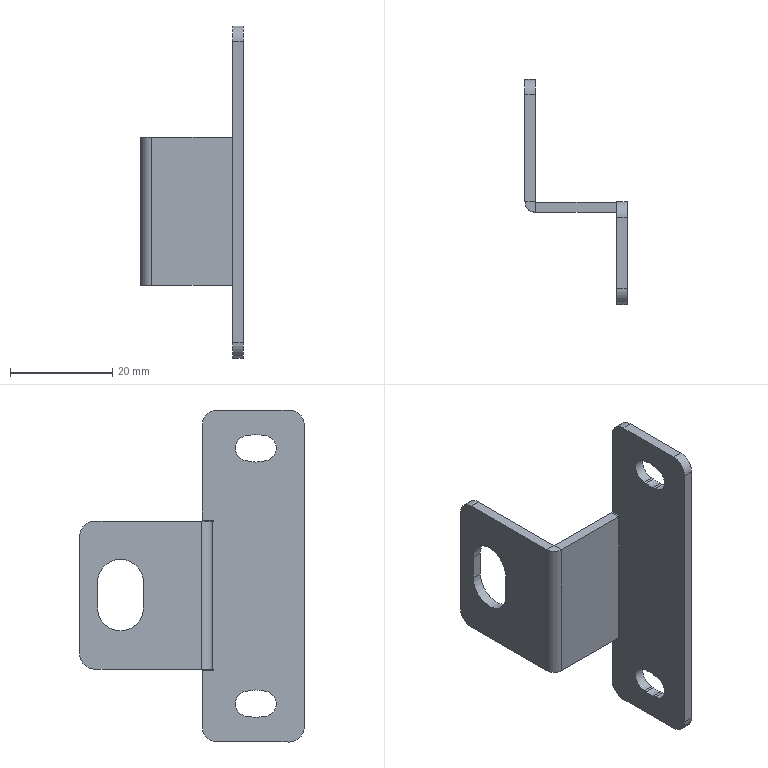Component | SolidWorks | RearDoorLockRodRetainer-1 | 1 solid | 59 faces | volume 4598 mm3 | plane 36 | cylinder 23 | commonest cylinder face diameters 5.4 x6 6 x6 5 x4 9 x3 4.2 x2 0.2 x2